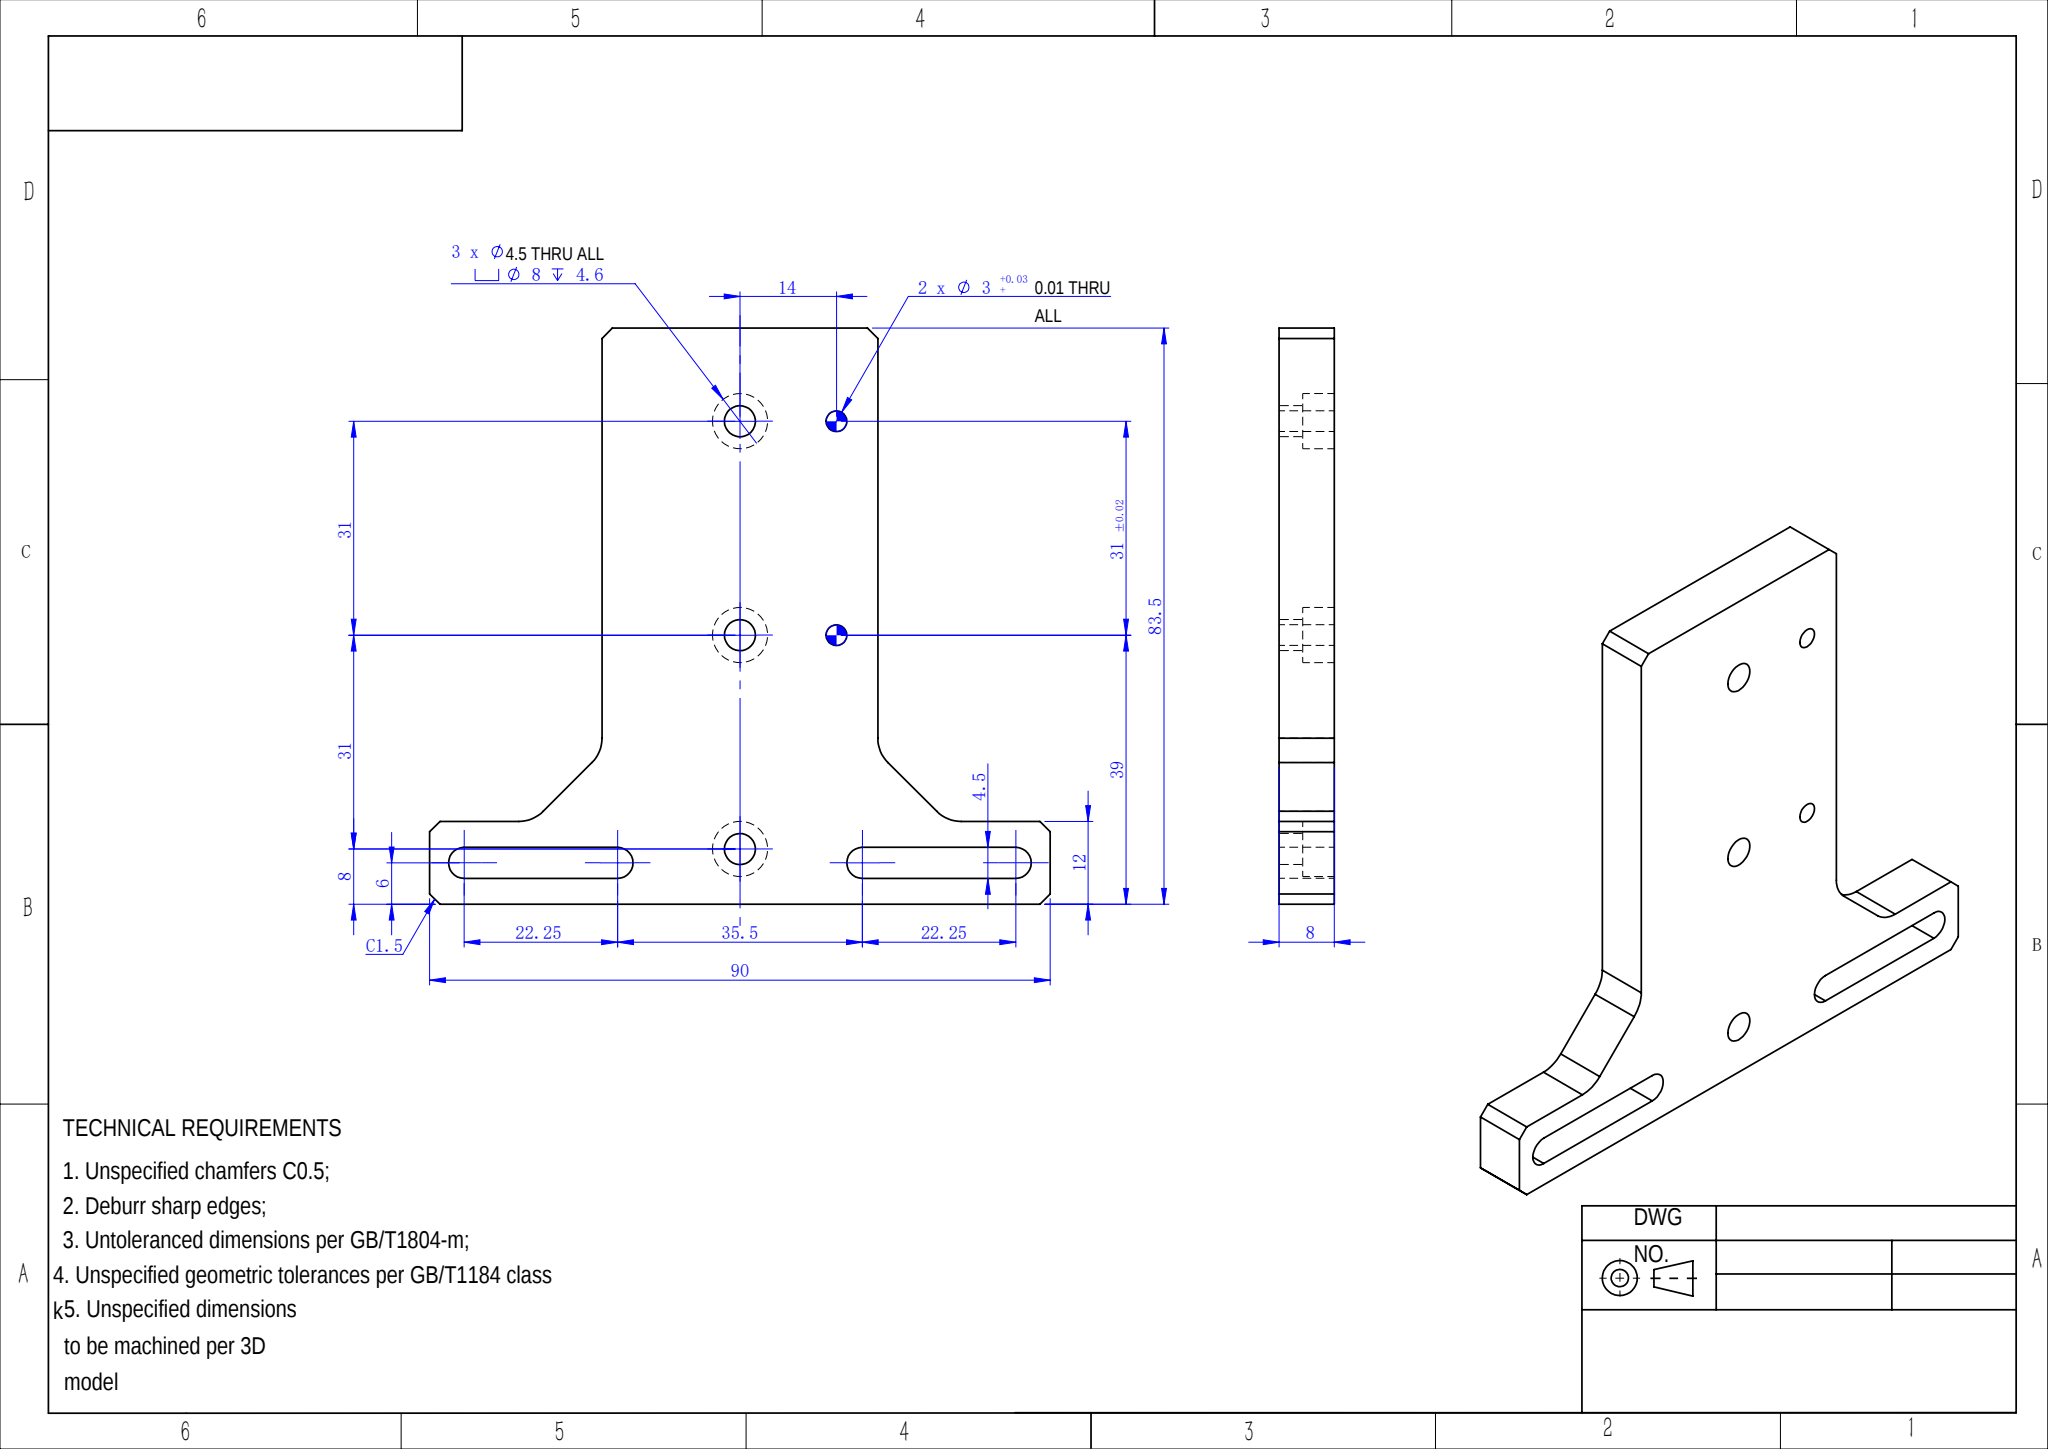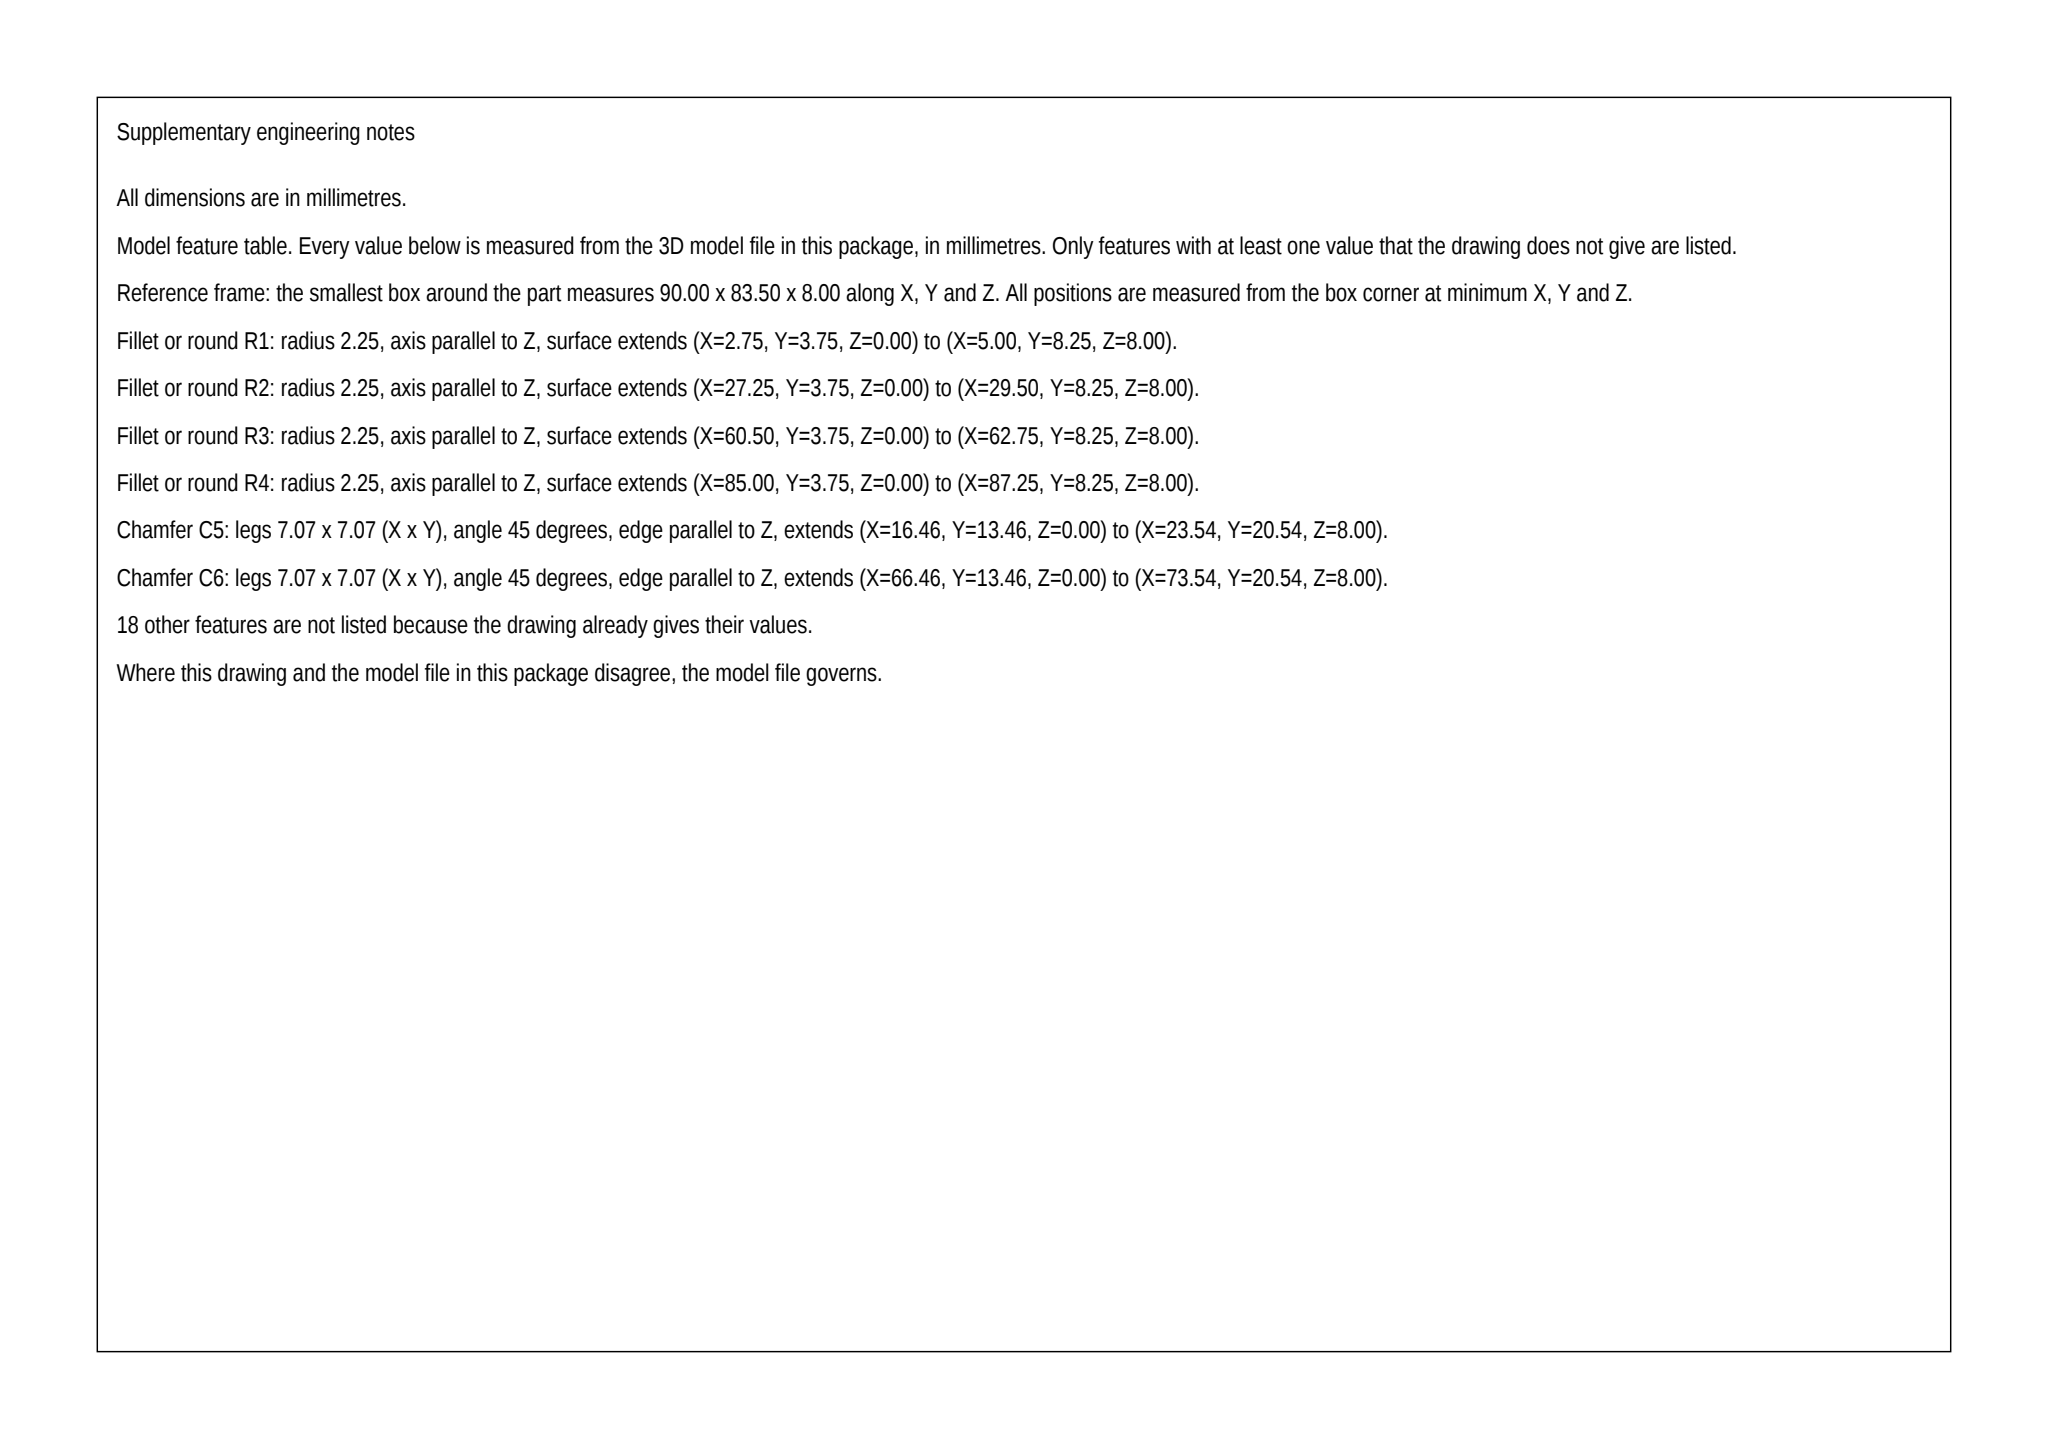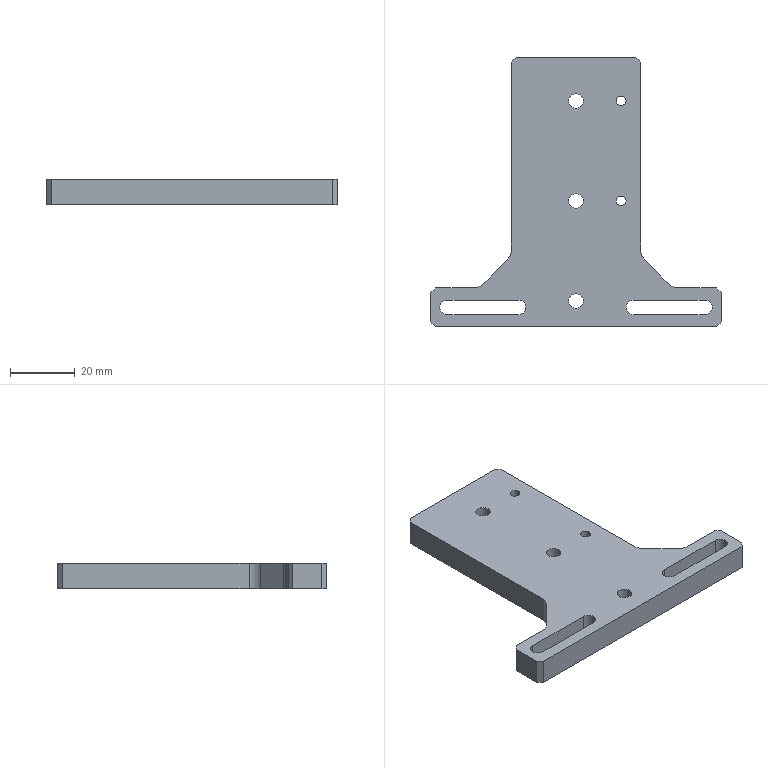Part | SolidWorks | mm | 1 solid | 51 faces | box 90 x 83.5 x 8 mm | volume 29458 mm3 | cylinder 26 | plane 25 | commonest cylinder face diameters 4.5 x12 8 x6 3 x4 10 x4
Drawing notes:
UPRIGHT PLATE 40 WIDE, SYM ABT HOLE CL; FACES 25 & 65 FROM LH EDGE | from the solid: x-planes at 25 and 65; hole axes x=45; bbox x=90
3X Ø4.5 THRU, CBORE Ø8 DP 4.6 FROM FRONT FACE | from the solid: Ø4.5 L3.4 coaxial with Ø8 L4.6 at x=45, y=8/39/70; z-plane 4.6
2X SLOT 4.5 W x 22.25 C-C THRU; END CTRS 5 FROM EACH SIDE EDGE, CL 6 UP | from the solid: Ø4.5 L8 cyls at (5,6),(27.25,6),(62.75,6),(85,6); y-planes 3.75 & 8.25
2X Ø3 CL 59 FROM LH EDGE, 14 FROM CBORE CL | from the solid: Ø3 thru cyls at x=59, y=39 & 70; cbore axes x=45
C1.5 2X BOTH BOTTOM CORNERS, SYM ABT CL 45 FROM LH EDGE | from the solid: base profile symmetric about x=45; bottom face y=0, sides x=0 and x=90
build123d program:
from build123d import *

# Parameters (mm, degrees)
SKETCH2_W                                         = 40
SKETCH2_H                                         = 83.5
BOSS_EXTRUDE1_DEPTH                               = 8
SKETCH3_W                                         = 25
SKETCH3_H                                         = 12
BOSS_EXTRUDE2_DEPTH                               = 8
CUT_EXTRUDE1_DEPTH                                = 62.904
CHAMFER1_SIZE                                     = 10
FILLET1_R                                         = 5
HOLE_SIZE_ACCORDING_TO_TYPE_1_OF_HEXA_D           = 4.5
HOLE_SIZE_ACCORDING_TO_TYPE_1_OF_HEXA_CBORE_D     = 8
HOLE_SIZE_ACCORDING_TO_TYPE_1_OF_HEXA_CBORE_DEPTH = 4.6
SIZE_MM_DOWEL_PIN_HOLE1_D                         = 3
CHAMFER2_SIZE                                     = 1.5


with BuildPart() as part:
    # Sketch2 → Boss-Extrude1 (new body)
    with BuildSketch(Plane.XY):
        Rectangle(SKETCH2_W, SKETCH2_H)
    extrude(amount=BOSS_EXTRUDE1_DEPTH)

    # Sketch3 → Boss-Extrude2 (add)
    with BuildSketch(Plane.XY.offset(8)):
        with Locations((32.5, -35.75)):
            Rectangle(SKETCH3_W, SKETCH3_H)
        with Locations((-32.5, -35.75)):
            Rectangle(SKETCH3_W, SKETCH3_H)
    extrude(amount=-BOSS_EXTRUDE2_DEPTH)

    # Sketch4 → Cut-Extrude1 (cut, through all)
    with BuildSketch(Plane.XY.offset(8)):
        with BuildLine():
            Line((17.75, -33.5), (40, -33.5))
            ThreePointArc((40, -33.5), (42.25, -35.75), (40, -38))
            Line((40, -38), (17.75, -38))
            ThreePointArc((17.75, -38), (15.5, -35.75), (17.75, -33.5))
        make_face()
        with BuildLine():
            Line((-17.75, -33.5), (-40, -33.5))
            ThreePointArc((-40, -33.5), (-42.25, -35.75), (-40, -38))
            Line((-40, -38), (-17.75, -38))
            ThreePointArc((-17.75, -38), (-15.5, -35.75), (-17.75, -33.5))
        make_face()
    extrude(amount=-CUT_EXTRUDE1_DEPTH, mode=Mode.SUBTRACT)

    # Chamfer1
    chamfer1_edges = [part.edges().sort_by_distance(p)[0] for p in [
        (20, -29.75, 4),
        (-20, -29.75, 4),
    ]]
    chamfer(chamfer1_edges, length=CHAMFER1_SIZE)

    # Fillet1
    fillet1_edges = [part.edges().sort_by_distance(p)[0] for p in [
        (-20, -19.75, 4),
        (-30, -29.75, 4),
        (30, -29.75, 4),
        (20, -19.75, 4),
    ]]
    fillet(fillet1_edges, radius=FILLET1_R)

    # Hole Size _ According to_ Type 1 of Hexa (through all)
    with Locations(Plane(origin=(0, 0, 0), x_dir=(-1, 0, 0), z_dir=(0, 0, -1))):
        with Locations((0, 28.25), (0, -2.75), (0, -33.75)):
            CounterBoreHole(HOLE_SIZE_ACCORDING_TO_TYPE_1_OF_HEXA_D / 2, HOLE_SIZE_ACCORDING_TO_TYPE_1_OF_HEXA_CBORE_D / 2, HOLE_SIZE_ACCORDING_TO_TYPE_1_OF_HEXA_CBORE_DEPTH)

    # Size mm Dowel Pin Hole1 (through all)
    with Locations(Plane(origin=(0, 0, 0), x_dir=(-1, 0, 0), z_dir=(0, 0, -1))):
        with Locations((-14, 28.25), (-14, -2.75)):
            Hole(SIZE_MM_DOWEL_PIN_HOLE1_D / 2)

    # Chamfer2
    chamfer2_edges = [part.edges().sort_by_distance(p)[0] for p in [
        (45, -41.75, 4),
        (45, -29.75, 4),
        (-45, -29.75, 4),
        (-45, -41.75, 4),
        (-20, 41.75, 4),
        (20, 41.75, 4),
    ]]
    chamfer(chamfer2_edges, length=CHAMFER2_SIZE)


solid = part.part